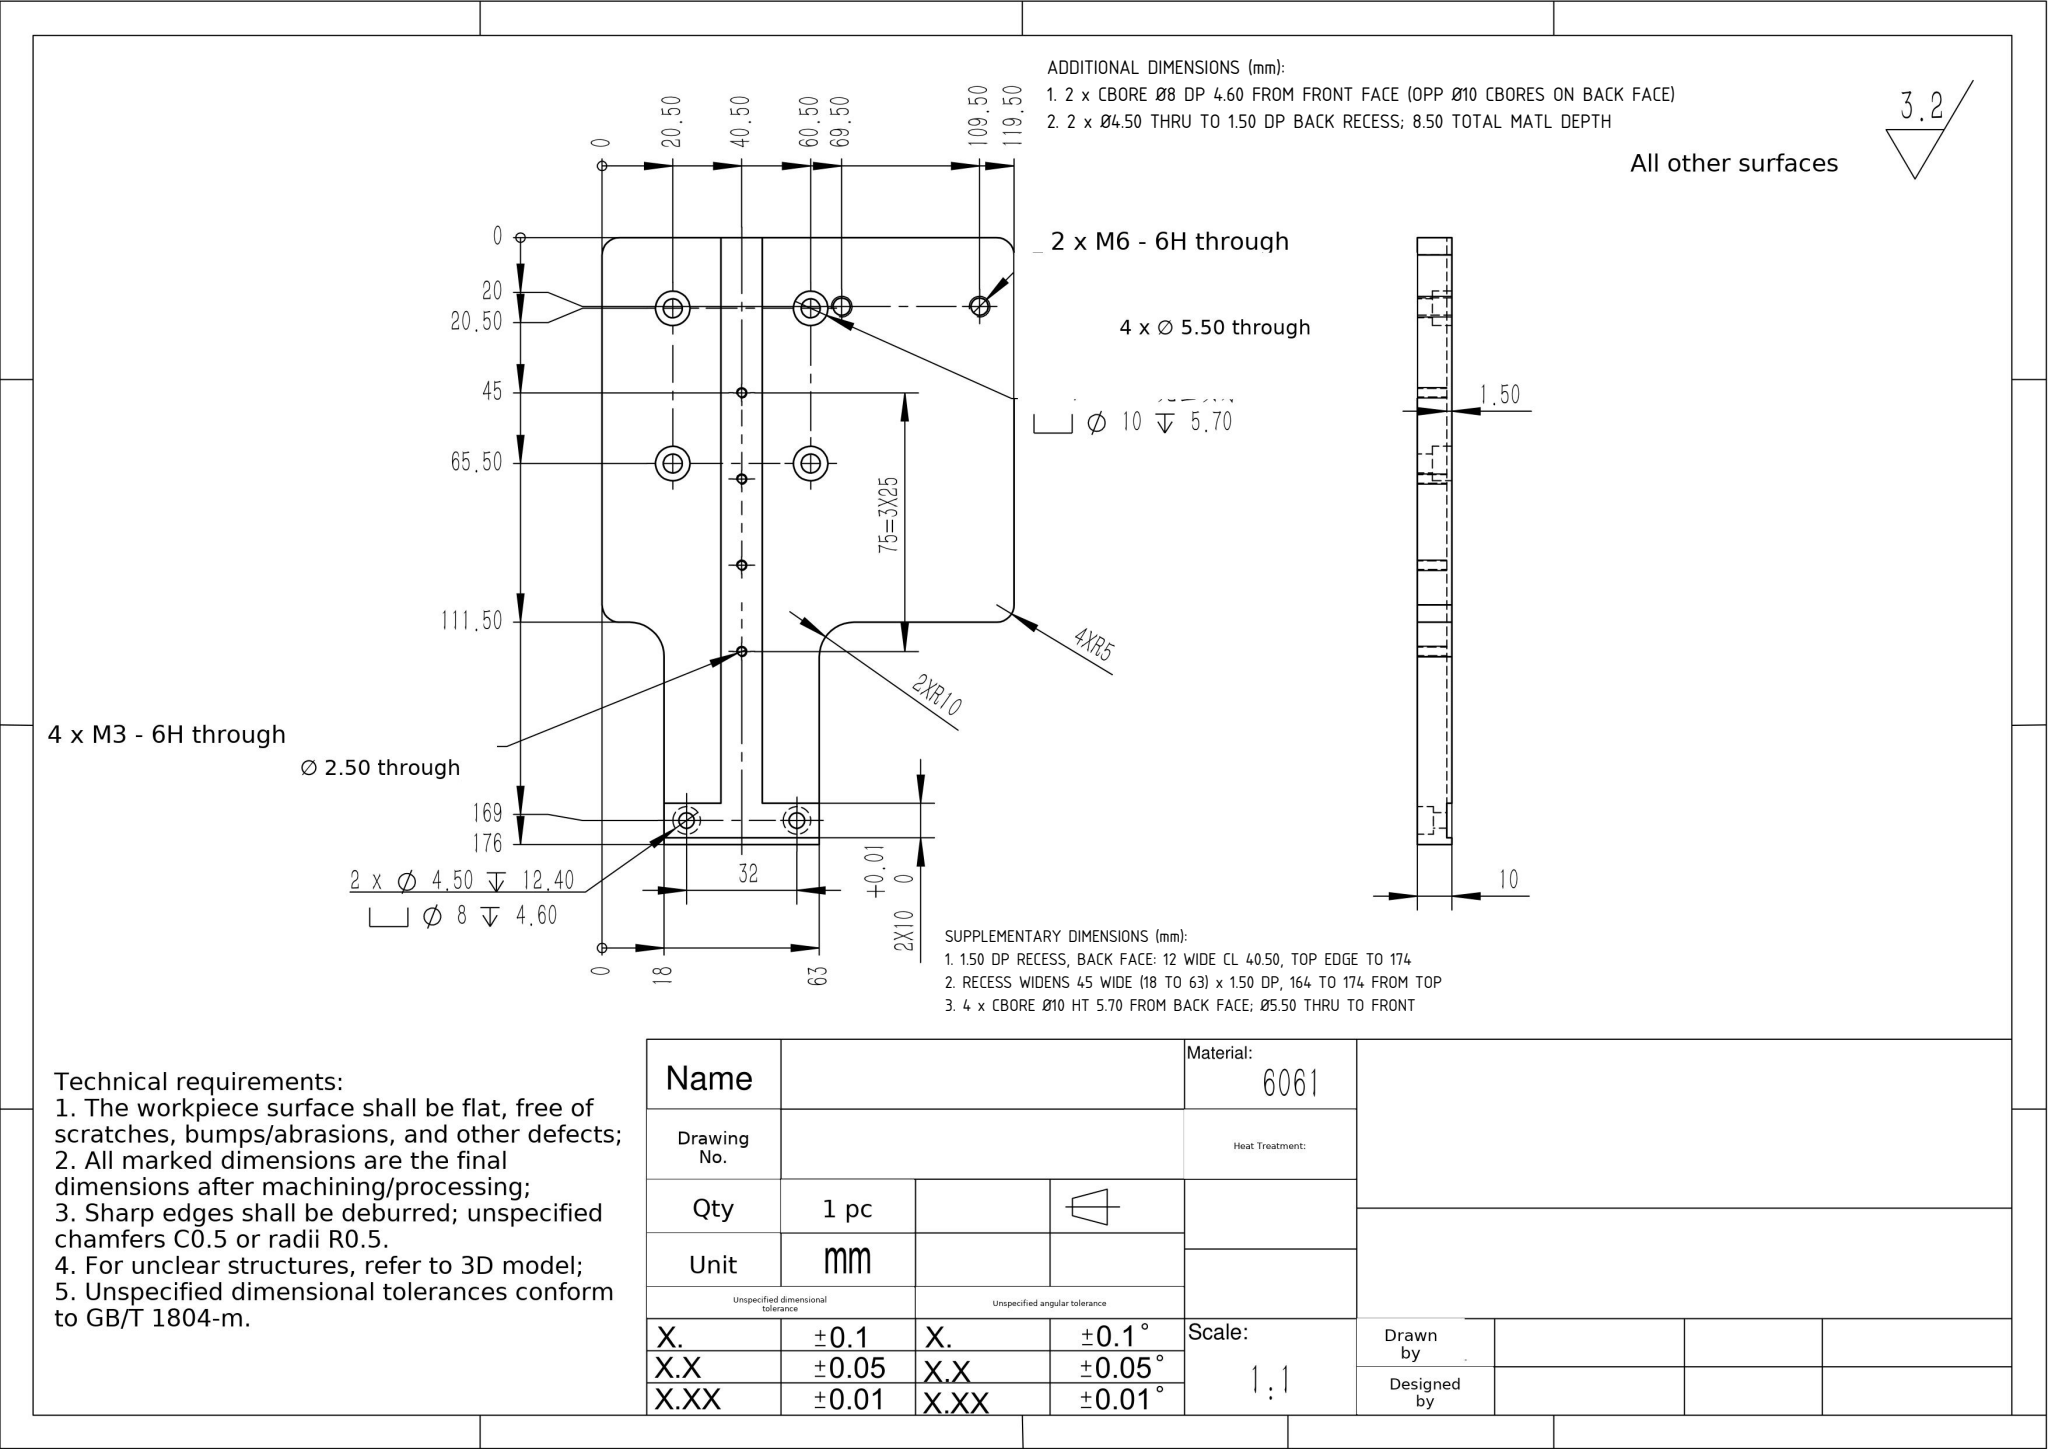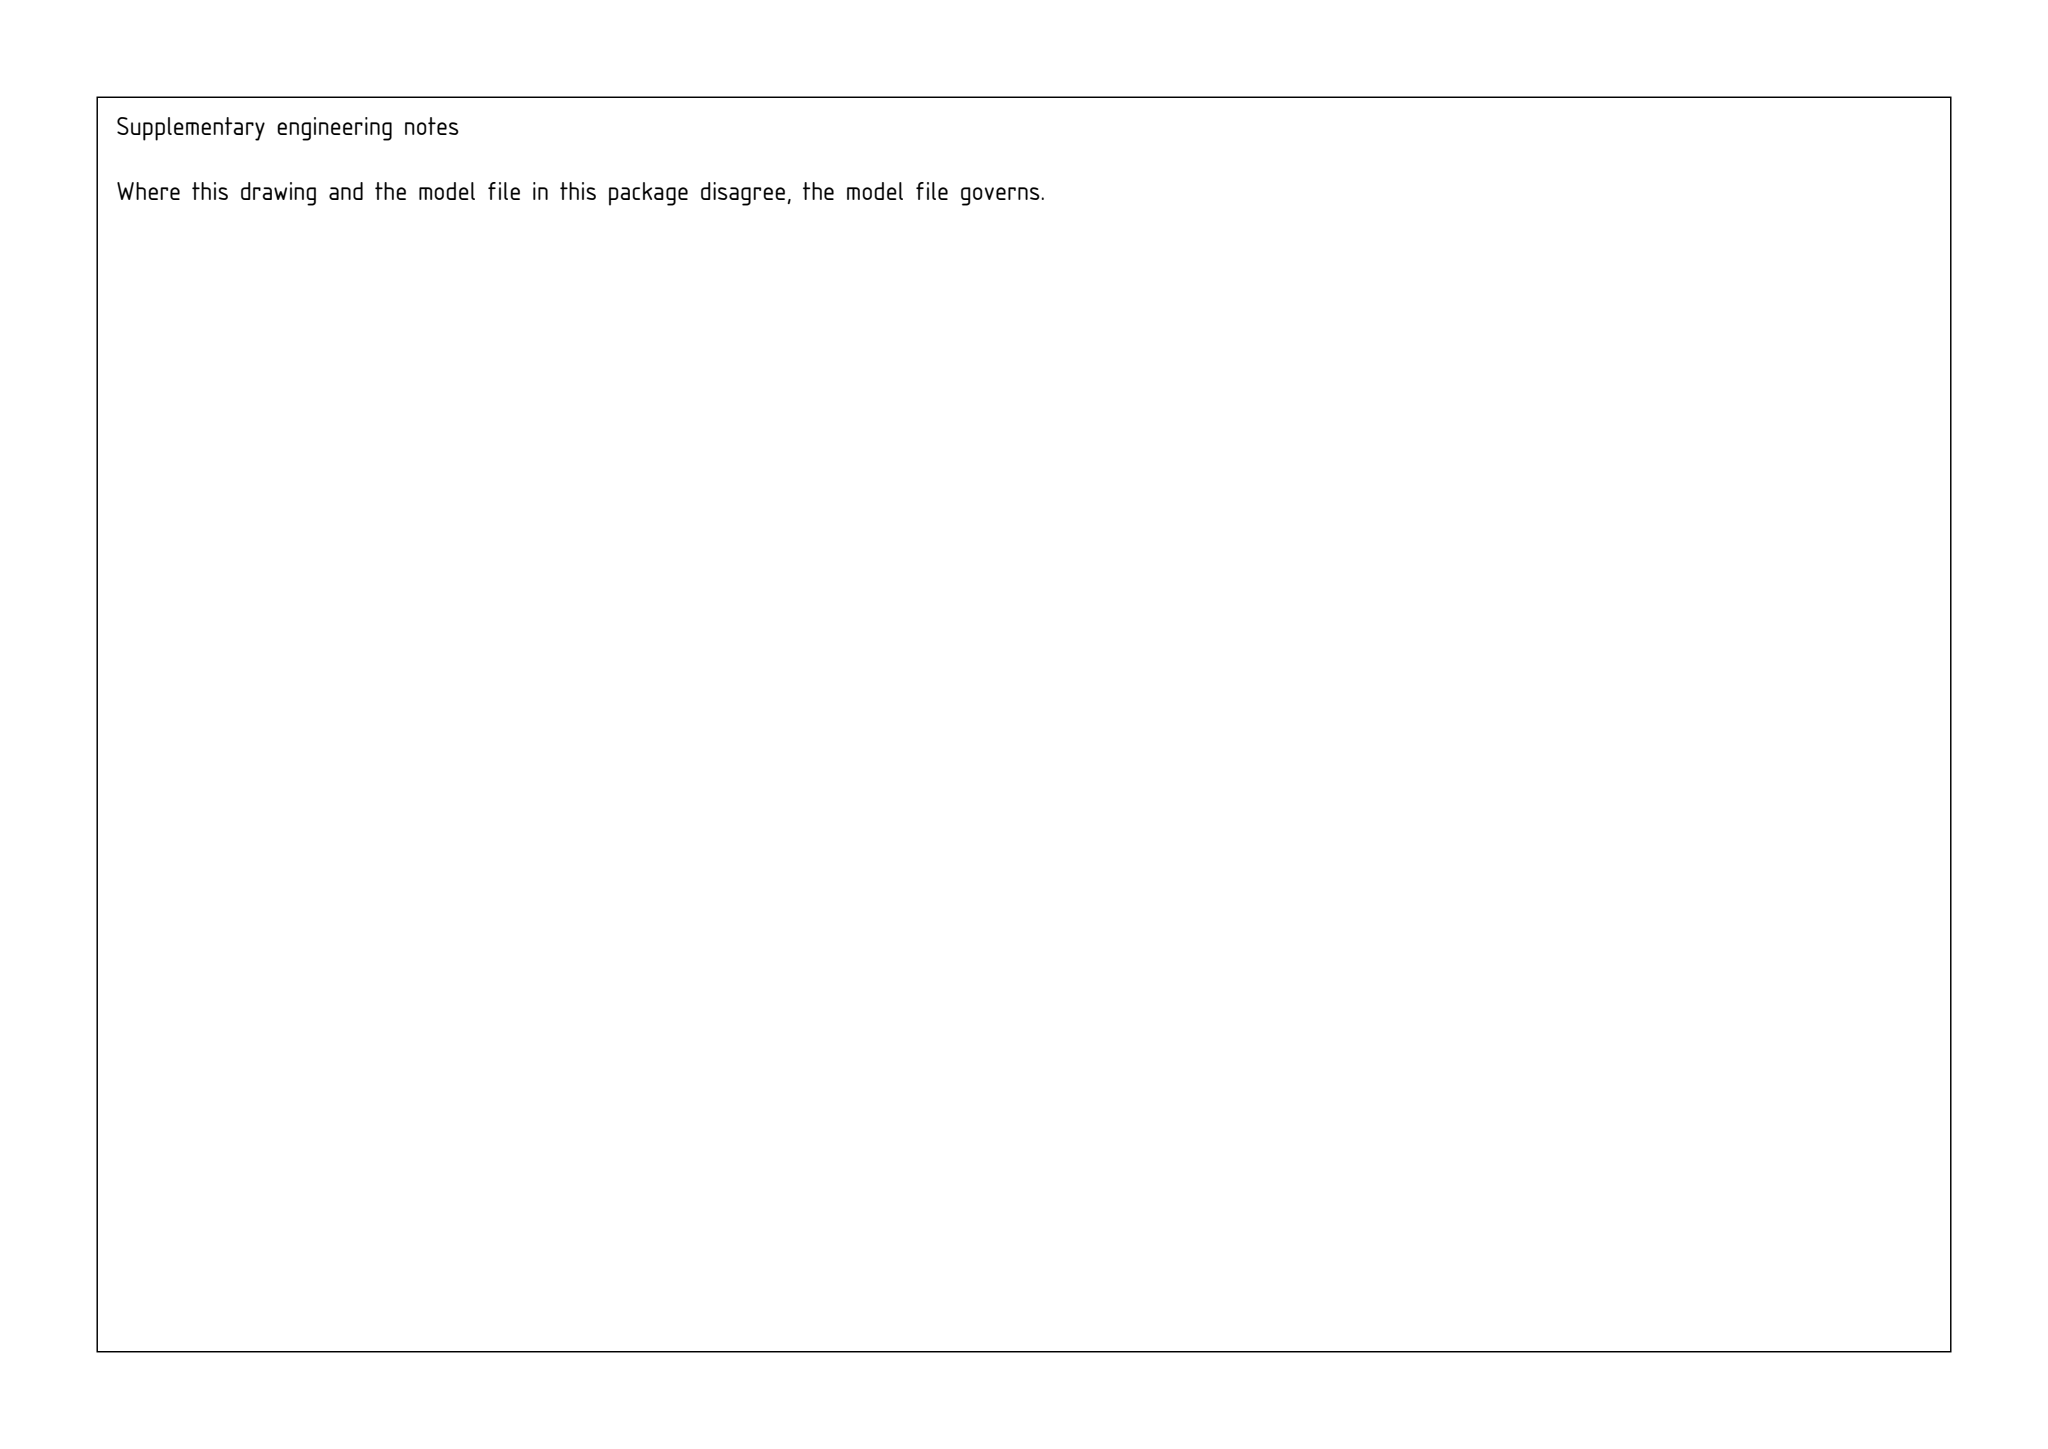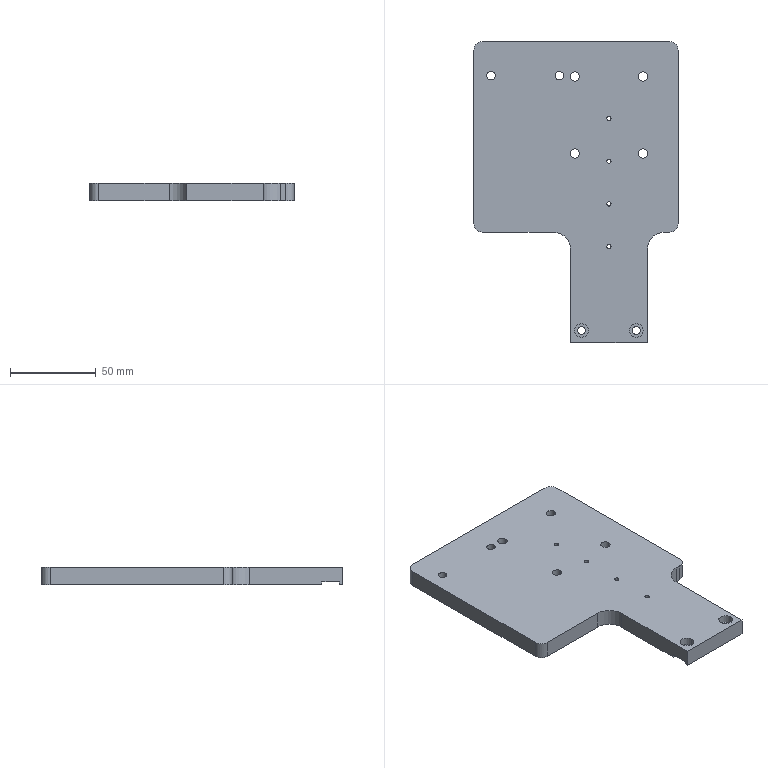Part | SolidWorks | mm | 1 solid | 66 faces | box 119.5 x 176 x 10 mm | volume 155510 mm3 | cylinder 42 | plane 24 | commonest cylinder face diameters 10 x12 5.5 x8 2.5 x8 5 x4 8 x4 4.5 x4 20 x2
build123d program:
from build123d import *

# Parameters (mm, degrees)
BOSS_EXTRUDE1_DEPTH                               = 10
CUT_EXTRUDE1_DEPTH                                = 1.5
HOLE_SIZE_ACCORDING_TO_TYPE_1_OF_HEXA_D           = 4.5
HOLE_SIZE_ACCORDING_TO_TYPE_1_OF_HEXA_DEPTH       = 12.4
HOLE_SIZE_ACCORDING_TO_TYPE_1_OF_HEXA_CBORE_D     = 8
HOLE_SIZE_ACCORDING_TO_TYPE_1_OF_HEXA_CBORE_DEPTH = 4.6
HOLE_SIZE_ACCORDING_TO_TYPE_1_OF_HEXA_TIP         = 1.352
M3_TAPPED_HOLE1_D                                 = 2.5
HOLE_SIZE_ACCORDING_TO_TYPE_2_OF_HEXA_D           = 5.5
HOLE_SIZE_ACCORDING_TO_TYPE_2_OF_HEXA_CBORE_D     = 10
HOLE_SIZE_ACCORDING_TO_TYPE_2_OF_HEXA_CBORE_DEPTH = 5.7
M6_TAPPED_HOLE1_D                                 = 5


with BuildPart() as part:
    # Sketch1 → Boss-Extrude1 (new body)
    with BuildSketch(Plane.XY):
        with BuildLine():
            Line((-54.75, -111.5), (-13.25, -111.5))
            ThreePointArc((-13.25, -111.5), (-6.179, -114.429), (-3.25, -121.5))
            Line((-3.25, -121.5), (-3.25, -176))
            Line((-3.25, -176), (41.75, -176))
            Line((41.75, -176), (41.75, -121.5))
            ThreePointArc((41.75, -121.5), (44.679, -114.429), (51.75, -111.5))
            Line((51.75, -111.5), (54.75, -111.5))
            ThreePointArc((54.75, -111.5), (58.286, -110.036), (59.75, -106.5))
            Line((59.75, -106.5), (59.75, -5))
            ThreePointArc((59.75, -5), (58.286, -1.464), (54.75, 0))
            Line((54.75, 0), (-54.75, 0))
            ThreePointArc((-54.75, 0), (-58.286, -1.464), (-59.75, -5))
            Line((-59.75, -5), (-59.75, -106.5))
            ThreePointArc((-59.75, -106.5), (-58.286, -110.036), (-54.75, -111.5))
        make_face()
    extrude(amount=BOSS_EXTRUDE1_DEPTH)

    # Sketch2 → Cut-Extrude1 (cut)
    with BuildSketch(Plane(origin=(0, 0, 0), x_dir=(-1, 0, 0), z_dir=(0, 0, -1))):
        Polygon((-25.25, 0), (-13.25, 0), (-13.25, -164), (3.25, -164), (3.25, -174), (-41.75, -174), (-41.75, -164), (-25.25, -164), align=None)
    extrude(amount=-CUT_EXTRUDE1_DEPTH, mode=Mode.SUBTRACT)

    # Hole Size _ according to_ Type 1 of Hexa
    with Locations(Plane(origin=(3.25, -169, 10), x_dir=(1, 0, 0), z_dir=(0, 0, 1))):
        with Locations((0, 0), (32, 0)):
            CounterBoreHole(HOLE_SIZE_ACCORDING_TO_TYPE_1_OF_HEXA_D / 2, HOLE_SIZE_ACCORDING_TO_TYPE_1_OF_HEXA_CBORE_D / 2, HOLE_SIZE_ACCORDING_TO_TYPE_1_OF_HEXA_CBORE_DEPTH, depth=HOLE_SIZE_ACCORDING_TO_TYPE_1_OF_HEXA_DEPTH)
            with Locations((0, 0, -(HOLE_SIZE_ACCORDING_TO_TYPE_1_OF_HEXA_DEPTH + HOLE_SIZE_ACCORDING_TO_TYPE_1_OF_HEXA_TIP / 2))):  # 118° drill point
                Cone(0, HOLE_SIZE_ACCORDING_TO_TYPE_1_OF_HEXA_D / 2, HOLE_SIZE_ACCORDING_TO_TYPE_1_OF_HEXA_TIP, mode=Mode.SUBTRACT)

    # M3 Tapped Hole1 (through all)
    with Locations(Plane(origin=(19.25, -120, 1.5), x_dir=(-1, 0, 0), z_dir=(0, 0, -1))):
        with Locations((0, 0), (0, 25), (0, 50), (0, 75)):
            Hole(M3_TAPPED_HOLE1_D / 2)

    # Hole Size _ according to_ Type 2 of Hexa (through all)
    with Locations(Plane(origin=(39.25, -65.5, 0), x_dir=(-1, 0, 0), z_dir=(0, 0, -1))):
        with Locations((0, 0), (40, 0), (40, 45), (0, 45)):
            CounterBoreHole(HOLE_SIZE_ACCORDING_TO_TYPE_2_OF_HEXA_D / 2, HOLE_SIZE_ACCORDING_TO_TYPE_2_OF_HEXA_CBORE_D / 2, HOLE_SIZE_ACCORDING_TO_TYPE_2_OF_HEXA_CBORE_DEPTH)

    # M6 Tapped Hole1 (through all)
    with Locations(Plane(origin=(-9.75, -20, 0), x_dir=(-1, 0, 0), z_dir=(0, 0, -1))):
        with Locations((0, 0), (40, 0)):
            Hole(M6_TAPPED_HOLE1_D / 2)


solid = part.part